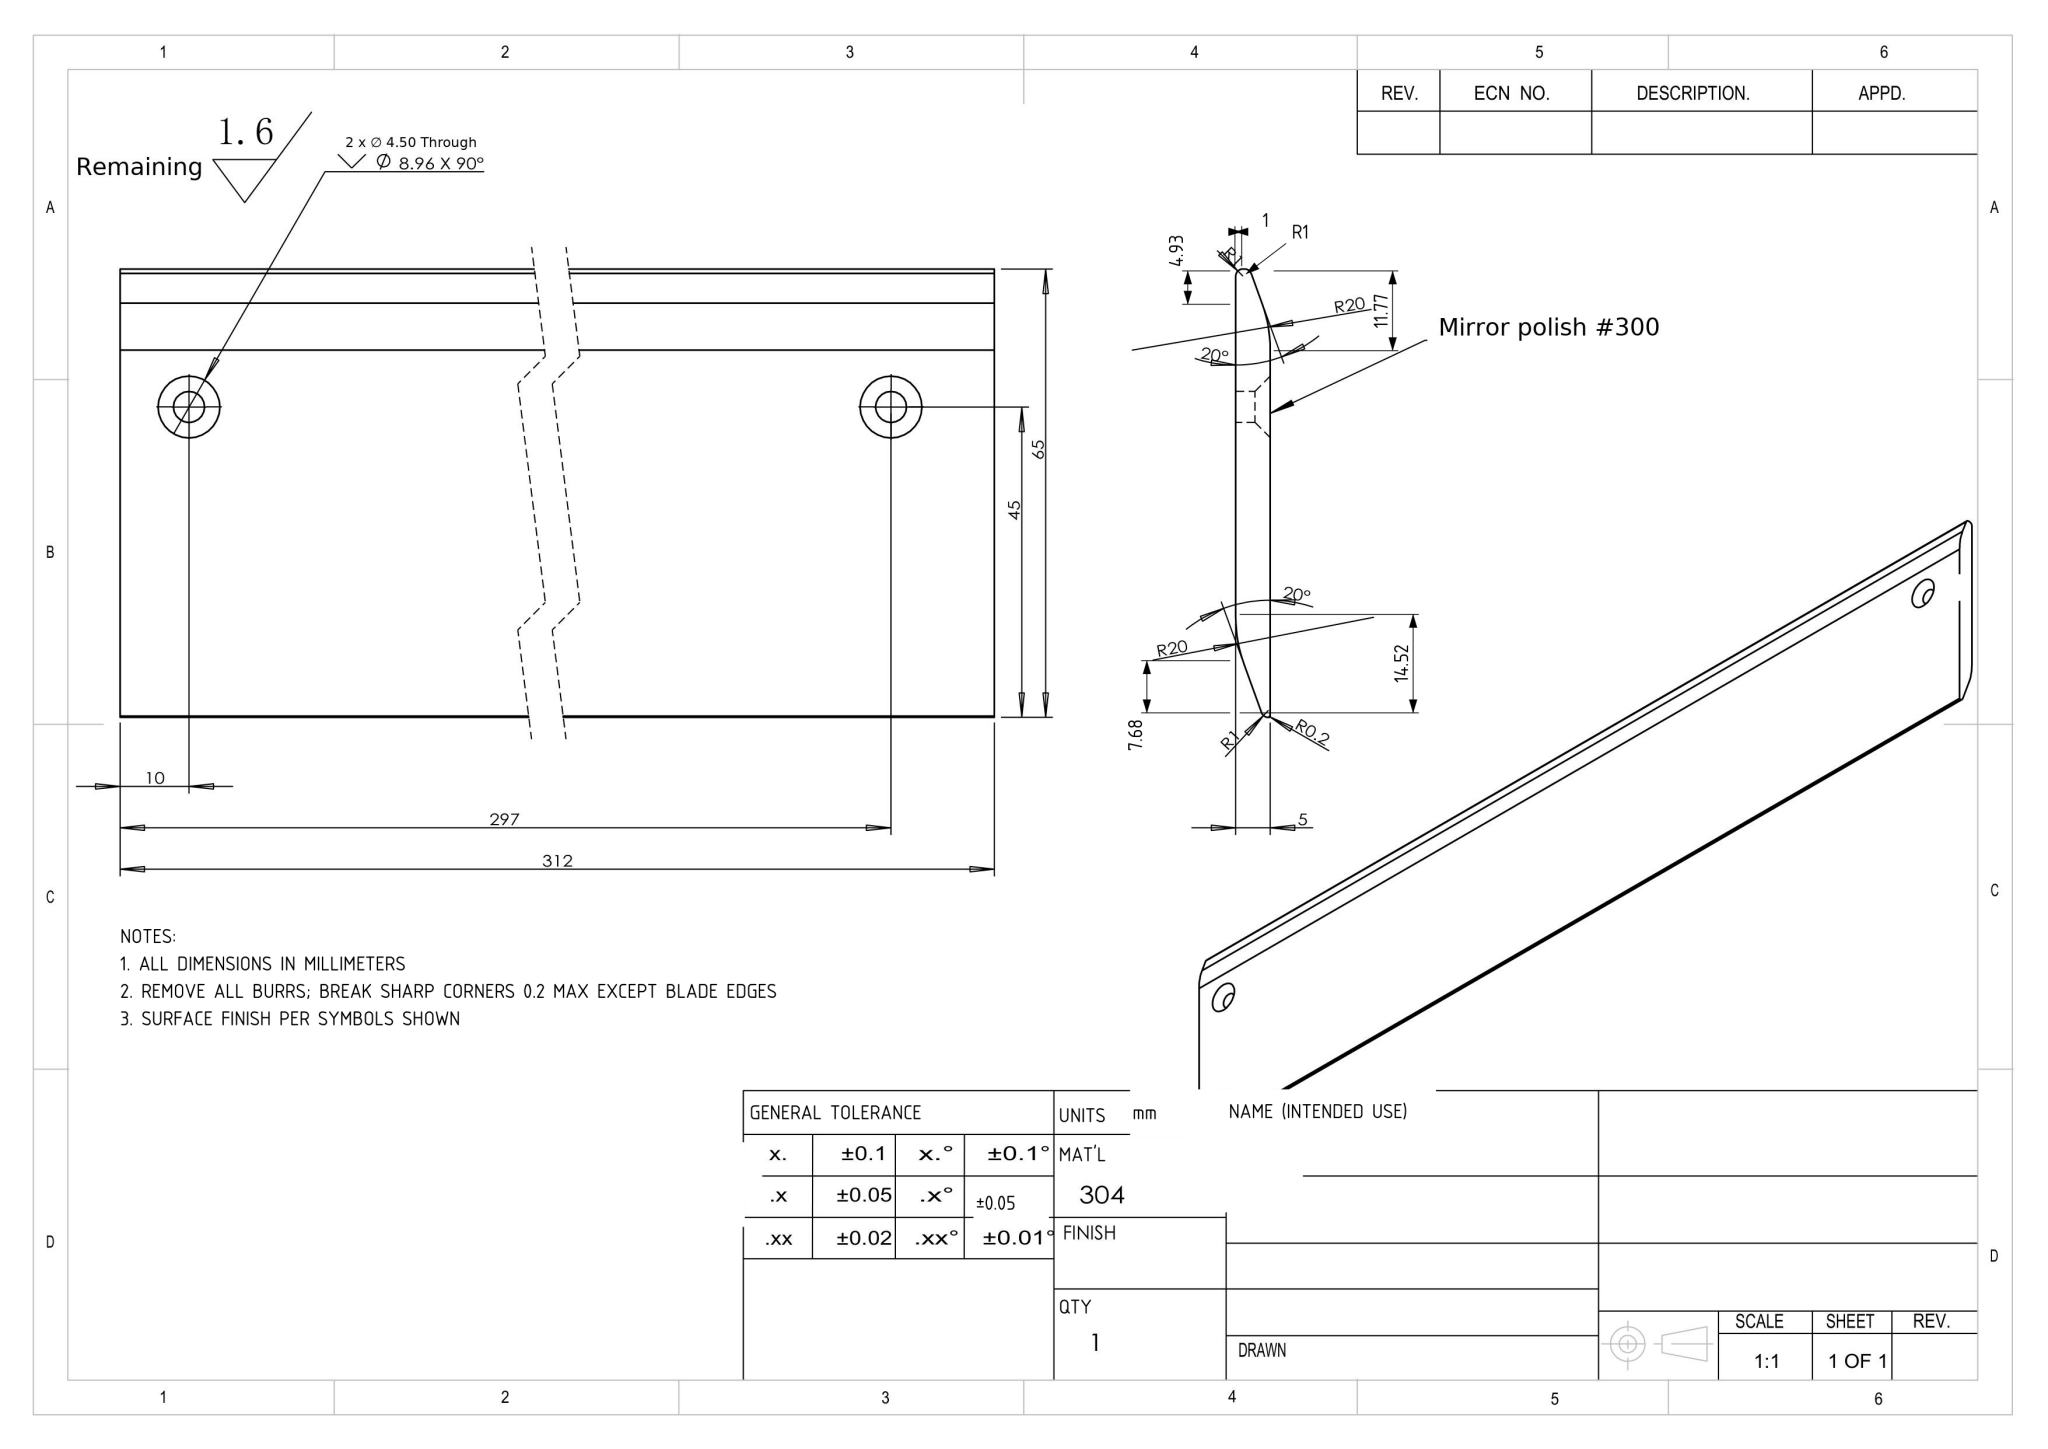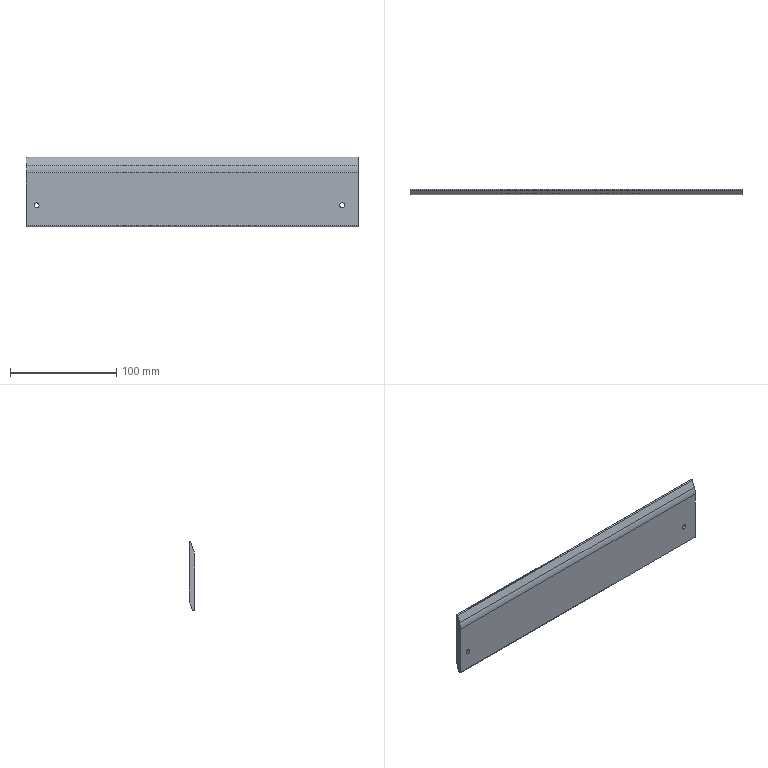Part | NX | mm | 1 solid | 22 faces | box 312 x 5 x 65 mm | volume 89859 mm3 | cylinder 10 | plane 8 | cone 4 | commonest cylinder face diameters 4.5 x4 2 x3 40 x2 0.4 x1
STEP:
#1=CARTESIAN_POINT('',(297.,2.77,-47.25));
#2=VERTEX_POINT('',#1);
#3=CARTESIAN_POINT('',(297.,2.77,-42.75));
#4=VERTEX_POINT('',#3);
#5=CARTESIAN_POINT('',(297.,2.77,-45.));
#6=DIRECTION('',(0.,1.,0.));
#7=DIRECTION('',(0.,0.,1.));
#8=AXIS2_PLACEMENT_3D('',#5,#6,#7);
#9=CIRCLE('',#8,2.25);
#10=EDGE_CURVE('',#2,#4,#9,.T.);
#11=ORIENTED_EDGE('',*,*,#10,.F.);
#12=CARTESIAN_POINT('',(297.,5.,-49.48));
#13=VERTEX_POINT('',#12);
#14=CARTESIAN_POINT('',(297.,5.,-49.48));
#15=DIRECTION('',(0.,0.7071,-0.7071));
#16=VECTOR('',#15,1000.);
#17=LINE('',#14,#16);
#18=EDGE_CURVE('',#2,#13,#17,.T.);
#19=ORIENTED_EDGE('',*,*,#18,.T.);
#20=CARTESIAN_POINT('',(297.,5.,-40.52));
#21=VERTEX_POINT('',#20);
#22=CARTESIAN_POINT('',(297.,5.,-45.));
#23=DIRECTION('',(0.,1.,0.));
#24=DIRECTION('',(0.,0.,1.));
#25=AXIS2_PLACEMENT_3D('',#22,#23,#24);
#26=CIRCLE('',#25,4.48);
#27=EDGE_CURVE('',#13,#21,#26,.T.);
#28=ORIENTED_EDGE('',*,*,#27,.T.);
#29=CARTESIAN_POINT('',(297.,5.,-40.52));
#30=DIRECTION('',(0.,0.7071,0.7071));
#31=VECTOR('',#30,1000.);
#32=LINE('',#29,#31);
#33=EDGE_CURVE('',#4,#21,#32,.T.);
#34=ORIENTED_EDGE('',*,*,#33,.F.);
#35=EDGE_LOOP('',(#11,#19,#28,#34));
#36=FACE_OUTER_BOUND('',#35,.T.);
#37=CARTESIAN_POINT('',(297.,5.,-45.));
#38=DIRECTION('',(0.,1.,0.));
#39=DIRECTION('',(0.,0.,1.));
#40=AXIS2_PLACEMENT_3D('',#37,#38,#39);
#41=CONICAL_SURFACE('',#40,4.48,0.7854);
#42=ADVANCED_FACE('',(#36),#41,.F.);
#43=CARTESIAN_POINT('',(297.,0.,-42.75));
#44=VERTEX_POINT('',#43);
#45=CARTESIAN_POINT('',(297.,0.,-47.25));
#46=VERTEX_POINT('',#45);
#47=CARTESIAN_POINT('',(297.,0.,-45.));
#48=DIRECTION('',(0.,-1.,0.));
#49=DIRECTION('',(0.,0.,-1.));
#50=AXIS2_PLACEMENT_3D('',#47,#48,#49);
#51=CIRCLE('',#50,2.25);
#52=EDGE_CURVE('',#44,#46,#51,.T.);
#53=ORIENTED_EDGE('',*,*,#52,.T.);
#54=CARTESIAN_POINT('',(297.,5.,-47.25));
#55=DIRECTION('',(0.,1.,0.));
#56=VECTOR('',#55,1000.);
#57=LINE('',#54,#56);
#58=EDGE_CURVE('',#46,#2,#57,.T.);
#59=ORIENTED_EDGE('',*,*,#58,.T.);
#60=ORIENTED_EDGE('',*,*,#10,.T.);
#61=CARTESIAN_POINT('',(297.,5.,-42.75));
#62=DIRECTION('',(0.,1.,0.));
#63=VECTOR('',#62,1000.);
#64=LINE('',#61,#63);
#65=EDGE_CURVE('',#44,#4,#64,.T.);
#66=ORIENTED_EDGE('',*,*,#65,.F.);
#67=EDGE_LOOP('',(#53,#59,#60,#66));
#68=FACE_OUTER_BOUND('',#67,.T.);
#69=CARTESIAN_POINT('',(297.,5.,-45.));
#70=DIRECTION('',(0.,1.,0.));
#71=DIRECTION('',(0.,0.,1.));
#72=AXIS2_PLACEMENT_3D('',#69,#70,#71);
#73=CYLINDRICAL_SURFACE('',#72,2.25);
#74=ADVANCED_FACE('',(#68),#73,.F.);
#75=CARTESIAN_POINT('',(10.,2.77,-47.25));
#76=VERTEX_POINT('',#75);
#77=CARTESIAN_POINT('',(10.,2.77,-42.75));
#78=VERTEX_POINT('',#77);
#79=CARTESIAN_POINT('',(10.,2.77,-45.));
#80=DIRECTION('',(0.,1.,0.));
#81=DIRECTION('',(0.,0.,1.));
#82=AXIS2_PLACEMENT_3D('',#79,#80,#81);
#83=CIRCLE('',#82,2.25);
#84=EDGE_CURVE('',#76,#78,#83,.T.);
#85=ORIENTED_EDGE('',*,*,#84,.F.);
#86=CARTESIAN_POINT('',(10.,5.,-49.48));
#87=VERTEX_POINT('',#86);
#88=CARTESIAN_POINT('',(10.,5.,-49.48));
#89=DIRECTION('',(0.,0.7071,-0.7071));
#90=VECTOR('',#89,1000.);
#91=LINE('',#88,#90);
#92=EDGE_CURVE('',#76,#87,#91,.T.);
#93=ORIENTED_EDGE('',*,*,#92,.T.);
#94=CARTESIAN_POINT('',(10.,5.,-40.52));
#95=VERTEX_POINT('',#94);
#96=CARTESIAN_POINT('',(10.,5.,-45.));
#97=DIRECTION('',(0.,1.,0.));
#98=DIRECTION('',(0.,0.,1.));
#99=AXIS2_PLACEMENT_3D('',#96,#97,#98);
#100=CIRCLE('',#99,4.48);
#101=EDGE_CURVE('',#87,#95,#100,.T.);
#102=ORIENTED_EDGE('',*,*,#101,.T.);
#103=CARTESIAN_POINT('',(10.,5.,-40.52));
#104=DIRECTION('',(0.,0.7071,0.7071));
#105=VECTOR('',#104,1000.);
#106=LINE('',#103,#105);
#107=EDGE_CURVE('',#78,#95,#106,.T.);
#108=ORIENTED_EDGE('',*,*,#107,.F.);
#109=EDGE_LOOP('',(#85,#93,#102,#108));
#110=FACE_OUTER_BOUND('',#109,.T.);
#111=CARTESIAN_POINT('',(10.,5.,-45.));
#112=DIRECTION('',(0.,1.,0.));
#113=DIRECTION('',(0.,0.,1.));
#114=AXIS2_PLACEMENT_3D('',#111,#112,#113);
#115=CONICAL_SURFACE('',#114,4.48,0.7854);
#116=ADVANCED_FACE('',(#110),#115,.F.);
#117=CARTESIAN_POINT('',(10.,0.,-42.75));
#118=VERTEX_POINT('',#117);
#119=CARTESIAN_POINT('',(10.,0.,-47.25));
#120=VERTEX_POINT('',#119);
#121=CARTESIAN_POINT('',(10.,0.,-45.));
#122=DIRECTION('',(0.,-1.,0.));
#123=DIRECTION('',(0.,0.,-1.));
#124=AXIS2_PLACEMENT_3D('',#121,#122,#123);
#125=CIRCLE('',#124,2.25);
#126=EDGE_CURVE('',#118,#120,#125,.T.);
#127=ORIENTED_EDGE('',*,*,#126,.T.);
#128=CARTESIAN_POINT('',(10.,5.,-47.25));
#129=DIRECTION('',(0.,1.,0.));
#130=VECTOR('',#129,1000.);
#131=LINE('',#128,#130);
#132=EDGE_CURVE('',#120,#76,#131,.T.);
#133=ORIENTED_EDGE('',*,*,#132,.T.);
#134=ORIENTED_EDGE('',*,*,#84,.T.);
#135=CARTESIAN_POINT('',(10.,5.,-42.75));
#136=DIRECTION('',(0.,1.,0.));
#137=VECTOR('',#136,1000.);
#138=LINE('',#135,#137);
#139=EDGE_CURVE('',#118,#78,#138,.T.);
#140=ORIENTED_EDGE('',*,*,#139,.F.);
#141=EDGE_LOOP('',(#127,#133,#134,#140));
#142=FACE_OUTER_BOUND('',#141,.T.);
#143=CARTESIAN_POINT('',(10.,5.,-45.));
#144=DIRECTION('',(0.,1.,0.));
#145=DIRECTION('',(0.,0.,1.));
#146=AXIS2_PLACEMENT_3D('',#143,#144,#145);
#147=CYLINDRICAL_SURFACE('',#146,2.25);
#148=ADVANCED_FACE('',(#142),#147,.F.);
#149=CARTESIAN_POINT('',(10.,5.,-45.));
#150=DIRECTION('',(0.,1.,0.));
#151=DIRECTION('',(0.,0.,1.));
#152=AXIS2_PLACEMENT_3D('',#149,#150,#151);
#153=CIRCLE('',#152,4.48);
#154=EDGE_CURVE('',#95,#87,#153,.T.);
#155=ORIENTED_EDGE('',*,*,#154,.F.);
#156=ORIENTED_EDGE('',*,*,#101,.F.);
#157=EDGE_LOOP('',(#155,#156));
#158=FACE_BOUND('',#157,.T.);
#159=CARTESIAN_POINT('',(0.,5.,-0.2));
#160=VERTEX_POINT('',#159);
#161=CARTESIAN_POINT('',(312.,5.,-0.2));
#162=VERTEX_POINT('',#161);
#163=CARTESIAN_POINT('',(0.,5.,-0.2));
#164=DIRECTION('',(1.,0.,0.));
#165=VECTOR('',#164,1000.);
#166=LINE('',#163,#165);
#167=EDGE_CURVE('',#160,#162,#166,.T.);
#168=ORIENTED_EDGE('',*,*,#167,.T.);
#169=CARTESIAN_POINT('',(312.,5.,-53.231));
#170=VERTEX_POINT('',#169);
#171=CARTESIAN_POINT('',(312.,5.,-0.));
#172=DIRECTION('',(0.,0.,1.));
#173=VECTOR('',#172,1000.);
#174=LINE('',#171,#173);
#175=EDGE_CURVE('',#170,#162,#174,.T.);
#176=ORIENTED_EDGE('',*,*,#175,.F.);
#177=CARTESIAN_POINT('',(0.,5.,-53.231));
#178=VERTEX_POINT('',#177);
#179=CARTESIAN_POINT('',(0.,5.,-53.231));
#180=DIRECTION('',(-1.,0.,0.));
#181=VECTOR('',#180,1000.);
#182=LINE('',#179,#181);
#183=EDGE_CURVE('',#170,#178,#182,.T.);
#184=ORIENTED_EDGE('',*,*,#183,.T.);
#185=CARTESIAN_POINT('',(0.,5.,0.));
#186=DIRECTION('',(0.,0.,1.));
#187=VECTOR('',#186,1000.);
#188=LINE('',#185,#187);
#189=EDGE_CURVE('',#178,#160,#188,.T.);
#190=ORIENTED_EDGE('',*,*,#189,.T.);
#191=EDGE_LOOP('',(#168,#176,#184,#190));
#192=FACE_OUTER_BOUND('',#191,.T.);
#193=CARTESIAN_POINT('',(297.,5.,-45.));
#194=DIRECTION('',(0.,1.,0.));
#195=DIRECTION('',(0.,0.,1.));
#196=AXIS2_PLACEMENT_3D('',#193,#194,#195);
#197=CIRCLE('',#196,4.48);
#198=EDGE_CURVE('',#21,#13,#197,.T.);
#199=ORIENTED_EDGE('',*,*,#198,.F.);
#200=ORIENTED_EDGE('',*,*,#27,.F.);
#201=EDGE_LOOP('',(#199,#200));
#202=FACE_BOUND('',#201,.T.);
#203=CARTESIAN_POINT('',(0.,5.,0.));
#204=DIRECTION('',(0.,-1.,0.));
#205=DIRECTION('',(0.,0.,-1.));
#206=AXIS2_PLACEMENT_3D('',#203,#204,#205);
#207=PLANE('',#206);
#208=ADVANCED_FACE('',(#158,#192,#202),#207,.F.);
#209=CARTESIAN_POINT('',(0.,4.8,0.));
#210=VERTEX_POINT('',#209);
#211=CARTESIAN_POINT('',(0.,4.7,0.));
#212=VERTEX_POINT('',#211);
#213=CARTESIAN_POINT('',(0.,5.,0.));
#214=DIRECTION('',(0.,-1.,0.));
#215=VECTOR('',#214,1000.);
#216=LINE('',#213,#215);
#217=EDGE_CURVE('',#210,#212,#216,.T.);
#218=ORIENTED_EDGE('',*,*,#217,.F.);
#219=CARTESIAN_POINT('',(0.,4.8,-0.2));
#220=DIRECTION('',(-1.,0.,0.));
#221=DIRECTION('',(0.,0.,-1.));
#222=AXIS2_PLACEMENT_3D('',#219,#220,#221);
#223=CIRCLE('',#222,0.2);
#224=EDGE_CURVE('',#210,#160,#223,.T.);
#225=ORIENTED_EDGE('',*,*,#224,.T.);
#226=ORIENTED_EDGE('',*,*,#189,.F.);
#227=CARTESIAN_POINT('',(0.,3.794,-60.071));
#228=VERTEX_POINT('',#227);
#229=CARTESIAN_POINT('',(0.,-15.,-53.231));
#230=DIRECTION('',(-1.,0.,0.));
#231=DIRECTION('',(0.,-0.,-1.));
#232=AXIS2_PLACEMENT_3D('',#229,#230,#231);
#233=CIRCLE('',#232,20.);
#234=EDGE_CURVE('',#178,#228,#233,.T.);
#235=ORIENTED_EDGE('',*,*,#234,.T.);
#236=CARTESIAN_POINT('',(0.,2.239,-64.342));
#237=VERTEX_POINT('',#236);
#238=CARTESIAN_POINT('',(0.,5.,-56.758));
#239=DIRECTION('',(0.,-0.342,-0.9397));
#240=VECTOR('',#239,1000.);
#241=LINE('',#238,#240);
#242=EDGE_CURVE('',#228,#237,#241,.T.);
#243=ORIENTED_EDGE('',*,*,#242,.T.);
#244=CARTESIAN_POINT('',(0.,1.3,-65.));
#245=VERTEX_POINT('',#244);
#246=CARTESIAN_POINT('',(0.,1.3,-64.));
#247=DIRECTION('',(-1.,0.,0.));
#248=DIRECTION('',(0.,0.,-1.));
#249=AXIS2_PLACEMENT_3D('',#246,#247,#248);
#250=CIRCLE('',#249,1.);
#251=EDGE_CURVE('',#237,#245,#250,.T.);
#252=ORIENTED_EDGE('',*,*,#251,.T.);
#253=CARTESIAN_POINT('',(0.,1.,-65.));
#254=VERTEX_POINT('',#253);
#255=CARTESIAN_POINT('',(0.,5.,-65.));
#256=DIRECTION('',(0.,-1.,0.));
#257=VECTOR('',#256,1000.);
#258=LINE('',#255,#257);
#259=EDGE_CURVE('',#245,#254,#258,.T.);
#260=ORIENTED_EDGE('',*,*,#259,.T.);
#261=CARTESIAN_POINT('',(0.,0.,-64.));
#262=VERTEX_POINT('',#261);
#263=CARTESIAN_POINT('',(0.,1.,-64.));
#264=DIRECTION('',(-1.,0.,0.));
#265=DIRECTION('',(0.,0.,-1.));
#266=AXIS2_PLACEMENT_3D('',#263,#264,#265);
#267=CIRCLE('',#266,1.);
#268=EDGE_CURVE('',#254,#262,#267,.T.);
#269=ORIENTED_EDGE('',*,*,#268,.T.);
#270=CARTESIAN_POINT('',(0.,0.,-14.516));
#271=VERTEX_POINT('',#270);
#272=CARTESIAN_POINT('',(0.,0.,0.));
#273=DIRECTION('',(0.,0.,1.));
#274=VECTOR('',#273,1000.);
#275=LINE('',#272,#274);
#276=EDGE_CURVE('',#262,#271,#275,.T.);
#277=ORIENTED_EDGE('',*,*,#276,.T.);
#278=CARTESIAN_POINT('',(0.,1.206,-7.676));
#279=VERTEX_POINT('',#278);
#280=CARTESIAN_POINT('',(0.,20.,-14.516));
#281=DIRECTION('',(-1.,0.,0.));
#282=DIRECTION('',(0.,0.,-1.));
#283=AXIS2_PLACEMENT_3D('',#280,#281,#282);
#284=CIRCLE('',#283,20.);
#285=EDGE_CURVE('',#271,#279,#284,.T.);
#286=ORIENTED_EDGE('',*,*,#285,.T.);
#287=CARTESIAN_POINT('',(0.,3.761,-0.658));
#288=VERTEX_POINT('',#287);
#289=CARTESIAN_POINT('',(0.,4.,0.));
#290=DIRECTION('',(0.,0.342,0.9397));
#291=VECTOR('',#290,1000.);
#292=LINE('',#289,#291);
#293=EDGE_CURVE('',#279,#288,#292,.T.);
#294=ORIENTED_EDGE('',*,*,#293,.T.);
#295=CARTESIAN_POINT('',(0.,4.7,-1.));
#296=DIRECTION('',(-1.,0.,0.));
#297=DIRECTION('',(0.,0.,-1.));
#298=AXIS2_PLACEMENT_3D('',#295,#296,#297);
#299=CIRCLE('',#298,1.);
#300=EDGE_CURVE('',#288,#212,#299,.T.);
#301=ORIENTED_EDGE('',*,*,#300,.T.);
#302=EDGE_LOOP('',(#218,#225,#226,#235,#243,#252,#260,#269,#277,#286,#294,#301));
#303=FACE_OUTER_BOUND('',#302,.T.);
#304=CARTESIAN_POINT('',(0.,5.,0.));
#305=DIRECTION('',(1.,0.,0.));
#306=DIRECTION('',(0.,0.,-1.));
#307=AXIS2_PLACEMENT_3D('',#304,#305,#306);
#308=PLANE('',#307);
#309=ADVANCED_FACE('',(#303),#308,.F.);
#310=CARTESIAN_POINT('',(312.,4.7,-0.));
#311=VERTEX_POINT('',#310);
#312=CARTESIAN_POINT('',(342.,4.7,0.));
#313=DIRECTION('',(1.,0.,0.));
#314=VECTOR('',#313,1000.);
#315=LINE('',#312,#314);
#316=EDGE_CURVE('',#212,#311,#315,.T.);
#317=ORIENTED_EDGE('',*,*,#316,.T.);
#318=CARTESIAN_POINT('',(312.,4.8,-0.));
#319=VERTEX_POINT('',#318);
#320=CARTESIAN_POINT('',(312.,-5.,-0.));
#321=DIRECTION('',(0.,1.,0.));
#322=VECTOR('',#321,1000.);
#323=LINE('',#320,#322);
#324=EDGE_CURVE('',#311,#319,#323,.T.);
#325=ORIENTED_EDGE('',*,*,#324,.T.);
#326=CARTESIAN_POINT('',(0.,4.8,0.));
#327=DIRECTION('',(-1.,0.,0.));
#328=VECTOR('',#327,1000.);
#329=LINE('',#326,#328);
#330=EDGE_CURVE('',#319,#210,#329,.T.);
#331=ORIENTED_EDGE('',*,*,#330,.T.);
#332=ORIENTED_EDGE('',*,*,#217,.T.);
#333=EDGE_LOOP('',(#317,#325,#331,#332));
#334=FACE_OUTER_BOUND('',#333,.T.);
#335=CARTESIAN_POINT('',(0.,5.,0.));
#336=DIRECTION('',(0.,0.,-1.));
#337=DIRECTION('',(-1.,0.,0.));
#338=AXIS2_PLACEMENT_3D('',#335,#336,#337);
#339=PLANE('',#338);
#340=ADVANCED_FACE('',(#334),#339,.F.);
#341=CARTESIAN_POINT('',(312.,1.3,-65.));
#342=VERTEX_POINT('',#341);
#343=CARTESIAN_POINT('',(342.,1.3,-65.));
#344=DIRECTION('',(1.,0.,0.));
#345=VECTOR('',#344,1000.);
#346=LINE('',#343,#345);
#347=EDGE_CURVE('',#245,#342,#346,.T.);
#348=ORIENTED_EDGE('',*,*,#347,.T.);
#349=CARTESIAN_POINT('',(312.,1.,-65.));
#350=VERTEX_POINT('',#349);
#351=CARTESIAN_POINT('',(312.,5.,-65.));
#352=DIRECTION('',(0.,-1.,0.));
#353=VECTOR('',#352,1000.);
#354=LINE('',#351,#353);
#355=EDGE_CURVE('',#342,#350,#354,.T.);
#356=ORIENTED_EDGE('',*,*,#355,.T.);
#357=CARTESIAN_POINT('',(0.,1.,-65.));
#358=DIRECTION('',(-1.,0.,0.));
#359=VECTOR('',#358,1000.);
#360=LINE('',#357,#359);
#361=EDGE_CURVE('',#350,#254,#360,.T.);
#362=ORIENTED_EDGE('',*,*,#361,.T.);
#363=ORIENTED_EDGE('',*,*,#259,.F.);
#364=EDGE_LOOP('',(#348,#356,#362,#363));
#365=FACE_OUTER_BOUND('',#364,.T.);
#366=CARTESIAN_POINT('',(0.,5.,-65.));
#367=DIRECTION('',(0.,0.,1.));
#368=DIRECTION('',(1.,0.,0.));
#369=AXIS2_PLACEMENT_3D('',#366,#367,#368);
#370=PLANE('',#369);
#371=ADVANCED_FACE('',(#365),#370,.F.);
#372=CARTESIAN_POINT('',(312.,0.,-14.516));
#373=VERTEX_POINT('',#372);
#374=CARTESIAN_POINT('',(312.,0.,-64.));
#375=VERTEX_POINT('',#374);
#376=CARTESIAN_POINT('',(312.,0.,0.));
#377=DIRECTION('',(0.,0.,-1.));
#378=VECTOR('',#377,1000.);
#379=LINE('',#376,#378);
#380=EDGE_CURVE('',#373,#375,#379,.T.);
#381=ORIENTED_EDGE('',*,*,#380,.F.);
#382=CARTESIAN_POINT('',(0.,0.,-14.516));
#383=DIRECTION('',(-1.,0.,0.));
#384=VECTOR('',#383,1000.);
#385=LINE('',#382,#384);
#386=EDGE_CURVE('',#373,#271,#385,.T.);
#387=ORIENTED_EDGE('',*,*,#386,.T.);
#388=ORIENTED_EDGE('',*,*,#276,.F.);
#389=CARTESIAN_POINT('',(342.,0.,-64.));
#390=DIRECTION('',(1.,0.,0.));
#391=VECTOR('',#390,1000.);
#392=LINE('',#389,#391);
#393=EDGE_CURVE('',#262,#375,#392,.T.);
#394=ORIENTED_EDGE('',*,*,#393,.T.);
#395=EDGE_LOOP('',(#381,#387,#388,#394));
#396=FACE_OUTER_BOUND('',#395,.T.);
#397=ORIENTED_EDGE('',*,*,#52,.F.);
#398=CARTESIAN_POINT('',(297.,0.,-45.));
#399=DIRECTION('',(0.,-1.,0.));
#400=DIRECTION('',(0.,0.,-1.));
#401=AXIS2_PLACEMENT_3D('',#398,#399,#400);
#402=CIRCLE('',#401,2.25);
#403=EDGE_CURVE('',#46,#44,#402,.T.);
#404=ORIENTED_EDGE('',*,*,#403,.F.);
#405=EDGE_LOOP('',(#397,#404));
#406=FACE_BOUND('',#405,.T.);
#407=ORIENTED_EDGE('',*,*,#126,.F.);
#408=CARTESIAN_POINT('',(10.,0.,-45.));
#409=DIRECTION('',(0.,-1.,0.));
#410=DIRECTION('',(0.,0.,-1.));
#411=AXIS2_PLACEMENT_3D('',#408,#409,#410);
#412=CIRCLE('',#411,2.25);
#413=EDGE_CURVE('',#120,#118,#412,.T.);
#414=ORIENTED_EDGE('',*,*,#413,.F.);
#415=EDGE_LOOP('',(#407,#414));
#416=FACE_BOUND('',#415,.T.);
#417=CARTESIAN_POINT('',(0.,0.,0.));
#418=DIRECTION('',(0.,-1.,0.));
#419=DIRECTION('',(0.,0.,-1.));
#420=AXIS2_PLACEMENT_3D('',#417,#418,#419);
#421=PLANE('',#420);
#422=ADVANCED_FACE('',(#396,#406,#416),#421,.T.);
#423=CARTESIAN_POINT('',(312.,2.239,-64.342));
#424=VERTEX_POINT('',#423);
#425=CARTESIAN_POINT('',(312.,3.794,-60.071));
#426=VERTEX_POINT('',#425);
#427=CARTESIAN_POINT('',(312.,5.,-56.758));
#428=DIRECTION('',(0.,0.342,0.9397));
#429=VECTOR('',#428,1000.);
#430=LINE('',#427,#429);
#431=EDGE_CURVE('',#424,#426,#430,.T.);
#432=ORIENTED_EDGE('',*,*,#431,.F.);
#433=CARTESIAN_POINT('',(0.,2.239,-64.342));
#434=DIRECTION('',(-1.,0.,0.));
#435=VECTOR('',#434,1000.);
#436=LINE('',#433,#435);
#437=EDGE_CURVE('',#424,#237,#436,.T.);
#438=ORIENTED_EDGE('',*,*,#437,.T.);
#439=ORIENTED_EDGE('',*,*,#242,.F.);
#440=CARTESIAN_POINT('',(342.,3.794,-60.071));
#441=DIRECTION('',(1.,0.,0.));
#442=VECTOR('',#441,1000.);
#443=LINE('',#440,#442);
#444=EDGE_CURVE('',#228,#426,#443,.T.);
#445=ORIENTED_EDGE('',*,*,#444,.T.);
#446=EDGE_LOOP('',(#432,#438,#439,#445));
#447=FACE_OUTER_BOUND('',#446,.T.);
#448=CARTESIAN_POINT('',(0.,5.,-56.758));
#449=DIRECTION('',(0.,-0.9397,0.342));
#450=DIRECTION('',(-1.,0.,0.));
#451=AXIS2_PLACEMENT_3D('',#448,#449,#450);
#452=PLANE('',#451);
#453=ADVANCED_FACE('',(#447),#452,.F.);
#454=CARTESIAN_POINT('',(312.,1.,-64.));
#455=DIRECTION('',(1.,0.,0.));
#456=DIRECTION('',(0.,0.,1.));
#457=AXIS2_PLACEMENT_3D('',#454,#455,#456);
#458=CIRCLE('',#457,1.);
#459=EDGE_CURVE('',#375,#350,#458,.T.);
#460=ORIENTED_EDGE('',*,*,#459,.F.);
#461=ORIENTED_EDGE('',*,*,#393,.F.);
#462=ORIENTED_EDGE('',*,*,#268,.F.);
#463=ORIENTED_EDGE('',*,*,#361,.F.);
#464=EDGE_LOOP('',(#460,#461,#462,#463));
#465=FACE_OUTER_BOUND('',#464,.T.);
#466=CARTESIAN_POINT('',(0.,1.,-64.));
#467=DIRECTION('',(1.,0.,0.));
#468=DIRECTION('',(0.,0.,-1.));
#469=AXIS2_PLACEMENT_3D('',#466,#467,#468);
#470=CYLINDRICAL_SURFACE('',#469,1.);
#471=ADVANCED_FACE('',(#465),#470,.T.);
#472=CARTESIAN_POINT('',(312.,1.3,-64.));
#473=DIRECTION('',(1.,0.,0.));
#474=DIRECTION('',(0.,0.,1.));
#475=AXIS2_PLACEMENT_3D('',#472,#473,#474);
#476=CIRCLE('',#475,1.);
#477=EDGE_CURVE('',#342,#424,#476,.T.);
#478=ORIENTED_EDGE('',*,*,#477,.F.);
#479=ORIENTED_EDGE('',*,*,#347,.F.);
#480=ORIENTED_EDGE('',*,*,#251,.F.);
#481=ORIENTED_EDGE('',*,*,#437,.F.);
#482=EDGE_LOOP('',(#478,#479,#480,#481));
#483=FACE_OUTER_BOUND('',#482,.T.);
#484=CARTESIAN_POINT('',(0.,1.3,-64.));
#485=DIRECTION('',(1.,0.,0.));
#486=DIRECTION('',(0.,0.,-1.));
#487=AXIS2_PLACEMENT_3D('',#484,#485,#486);
#488=CYLINDRICAL_SURFACE('',#487,1.);
#489=ADVANCED_FACE('',(#483),#488,.T.);
#490=CARTESIAN_POINT('',(312.,-15.,-53.231));
#491=DIRECTION('',(1.,0.,0.));
#492=DIRECTION('',(0.,-0.,1.));
#493=AXIS2_PLACEMENT_3D('',#490,#491,#492);
#494=CIRCLE('',#493,20.);
#495=EDGE_CURVE('',#426,#170,#494,.T.);
#496=ORIENTED_EDGE('',*,*,#495,.F.);
#497=ORIENTED_EDGE('',*,*,#444,.F.);
#498=ORIENTED_EDGE('',*,*,#234,.F.);
#499=ORIENTED_EDGE('',*,*,#183,.F.);
#500=EDGE_LOOP('',(#496,#497,#498,#499));
#501=FACE_OUTER_BOUND('',#500,.T.);
#502=CARTESIAN_POINT('',(0.,-15.,-53.231));
#503=DIRECTION('',(-1.,0.,0.));
#504=DIRECTION('',(0.,0.,1.));
#505=AXIS2_PLACEMENT_3D('',#502,#503,#504);
#506=CYLINDRICAL_SURFACE('',#505,20.);
#507=ADVANCED_FACE('',(#501),#506,.T.);
#508=ORIENTED_EDGE('',*,*,#132,.F.);
#509=ORIENTED_EDGE('',*,*,#413,.T.);
#510=ORIENTED_EDGE('',*,*,#139,.T.);
#511=CARTESIAN_POINT('',(10.,2.77,-45.));
#512=DIRECTION('',(0.,1.,0.));
#513=DIRECTION('',(0.,0.,1.));
#514=AXIS2_PLACEMENT_3D('',#511,#512,#513);
#515=CIRCLE('',#514,2.25);
#516=EDGE_CURVE('',#78,#76,#515,.T.);
#517=ORIENTED_EDGE('',*,*,#516,.T.);
#518=EDGE_LOOP('',(#508,#509,#510,#517));
#519=FACE_OUTER_BOUND('',#518,.T.);
#520=CARTESIAN_POINT('',(10.,5.,-45.));
#521=DIRECTION('',(0.,1.,0.));
#522=DIRECTION('',(0.,0.,1.));
#523=AXIS2_PLACEMENT_3D('',#520,#521,#522);
#524=CYLINDRICAL_SURFACE('',#523,2.25);
#525=ADVANCED_FACE('',(#519),#524,.F.);
#526=ORIENTED_EDGE('',*,*,#92,.F.);
#527=ORIENTED_EDGE('',*,*,#516,.F.);
#528=ORIENTED_EDGE('',*,*,#107,.T.);
#529=ORIENTED_EDGE('',*,*,#154,.T.);
#530=EDGE_LOOP('',(#526,#527,#528,#529));
#531=FACE_OUTER_BOUND('',#530,.T.);
#532=CARTESIAN_POINT('',(10.,5.,-45.));
#533=DIRECTION('',(0.,1.,0.));
#534=DIRECTION('',(0.,0.,1.));
#535=AXIS2_PLACEMENT_3D('',#532,#533,#534);
#536=CONICAL_SURFACE('',#535,4.48,0.7854);
#537=ADVANCED_FACE('',(#531),#536,.F.);
#538=ORIENTED_EDGE('',*,*,#58,.F.);
#539=ORIENTED_EDGE('',*,*,#403,.T.);
#540=ORIENTED_EDGE('',*,*,#65,.T.);
#541=CARTESIAN_POINT('',(297.,2.77,-45.));
#542=DIRECTION('',(0.,1.,0.));
#543=DIRECTION('',(0.,0.,1.));
#544=AXIS2_PLACEMENT_3D('',#541,#542,#543);
#545=CIRCLE('',#544,2.25);
#546=EDGE_CURVE('',#4,#2,#545,.T.);
#547=ORIENTED_EDGE('',*,*,#546,.T.);
#548=EDGE_LOOP('',(#538,#539,#540,#547));
#549=FACE_OUTER_BOUND('',#548,.T.);
#550=CARTESIAN_POINT('',(297.,5.,-45.));
#551=DIRECTION('',(0.,1.,0.));
#552=DIRECTION('',(0.,0.,1.));
#553=AXIS2_PLACEMENT_3D('',#550,#551,#552);
#554=CYLINDRICAL_SURFACE('',#553,2.25);
#555=ADVANCED_FACE('',(#549),#554,.F.);
#556=ORIENTED_EDGE('',*,*,#18,.F.);
#557=ORIENTED_EDGE('',*,*,#546,.F.);
#558=ORIENTED_EDGE('',*,*,#33,.T.);
#559=ORIENTED_EDGE('',*,*,#198,.T.);
#560=EDGE_LOOP('',(#556,#557,#558,#559));
#561=FACE_OUTER_BOUND('',#560,.T.);
#562=CARTESIAN_POINT('',(297.,5.,-45.));
#563=DIRECTION('',(0.,1.,0.));
#564=DIRECTION('',(0.,0.,1.));
#565=AXIS2_PLACEMENT_3D('',#562,#563,#564);
#566=CONICAL_SURFACE('',#565,4.48,0.7854);
#567=ADVANCED_FACE('',(#561),#566,.F.);
#568=CARTESIAN_POINT('',(312.,3.761,-0.658));
#569=VERTEX_POINT('',#568);
#570=CARTESIAN_POINT('',(312.,1.206,-7.676));
#571=VERTEX_POINT('',#570);
#572=CARTESIAN_POINT('',(312.,4.,0.));
#573=DIRECTION('',(0.,-0.342,-0.9397));
#574=VECTOR('',#573,1000.);
#575=LINE('',#572,#574);
#576=EDGE_CURVE('',#569,#571,#575,.T.);
#577=ORIENTED_EDGE('',*,*,#576,.F.);
#578=CARTESIAN_POINT('',(0.,3.761,-0.658));
#579=DIRECTION('',(-1.,0.,0.));
#580=VECTOR('',#579,1000.);
#581=LINE('',#578,#580);
#582=EDGE_CURVE('',#569,#288,#581,.T.);
#583=ORIENTED_EDGE('',*,*,#582,.T.);
#584=ORIENTED_EDGE('',*,*,#293,.F.);
#585=CARTESIAN_POINT('',(0.,1.206,-7.676));
#586=DIRECTION('',(1.,0.,0.));
#587=VECTOR('',#586,1000.);
#588=LINE('',#585,#587);
#589=EDGE_CURVE('',#279,#571,#588,.T.);
#590=ORIENTED_EDGE('',*,*,#589,.T.);
#591=EDGE_LOOP('',(#577,#583,#584,#590));
#592=FACE_OUTER_BOUND('',#591,.T.);
#593=CARTESIAN_POINT('',(0.,4.,0.));
#594=DIRECTION('',(0.,-0.9397,0.342));
#595=DIRECTION('',(-1.,0.,0.));
#596=AXIS2_PLACEMENT_3D('',#593,#594,#595);
#597=PLANE('',#596);
#598=ADVANCED_FACE('',(#592),#597,.T.);
#599=CARTESIAN_POINT('',(312.,20.,-14.516));
#600=DIRECTION('',(1.,0.,0.));
#601=DIRECTION('',(0.,0.,1.));
#602=AXIS2_PLACEMENT_3D('',#599,#600,#601);
#603=CIRCLE('',#602,20.);
#604=EDGE_CURVE('',#571,#373,#603,.T.);
#605=ORIENTED_EDGE('',*,*,#604,.F.);
#606=ORIENTED_EDGE('',*,*,#589,.F.);
#607=ORIENTED_EDGE('',*,*,#285,.F.);
#608=ORIENTED_EDGE('',*,*,#386,.F.);
#609=EDGE_LOOP('',(#605,#606,#607,#608));
#610=FACE_OUTER_BOUND('',#609,.T.);
#611=CARTESIAN_POINT('',(0.,20.,-14.516));
#612=DIRECTION('',(-1.,0.,0.));
#613=DIRECTION('',(0.,0.,1.));
#614=AXIS2_PLACEMENT_3D('',#611,#612,#613);
#615=CYLINDRICAL_SURFACE('',#614,20.);
#616=ADVANCED_FACE('',(#610),#615,.T.);
#617=CARTESIAN_POINT('',(312.,4.7,-1.));
#618=DIRECTION('',(1.,0.,0.));
#619=DIRECTION('',(0.,0.,1.));
#620=AXIS2_PLACEMENT_3D('',#617,#618,#619);
#621=CIRCLE('',#620,1.);
#622=EDGE_CURVE('',#311,#569,#621,.T.);
#623=ORIENTED_EDGE('',*,*,#622,.F.);
#624=ORIENTED_EDGE('',*,*,#316,.F.);
#625=ORIENTED_EDGE('',*,*,#300,.F.);
#626=ORIENTED_EDGE('',*,*,#582,.F.);
#627=EDGE_LOOP('',(#623,#624,#625,#626));
#628=FACE_OUTER_BOUND('',#627,.T.);
#629=CARTESIAN_POINT('',(0.,4.7,-1.));
#630=DIRECTION('',(-1.,0.,0.));
#631=DIRECTION('',(0.,0.,1.));
#632=AXIS2_PLACEMENT_3D('',#629,#630,#631);
#633=CYLINDRICAL_SURFACE('',#632,1.);
#634=ADVANCED_FACE('',(#628),#633,.T.);
#635=CARTESIAN_POINT('',(312.,4.8,-0.2));
#636=DIRECTION('',(1.,0.,0.));
#637=DIRECTION('',(0.,0.,1.));
#638=AXIS2_PLACEMENT_3D('',#635,#636,#637);
#639=CIRCLE('',#638,0.2);
#640=EDGE_CURVE('',#162,#319,#639,.T.);
#641=ORIENTED_EDGE('',*,*,#640,.F.);
#642=ORIENTED_EDGE('',*,*,#167,.F.);
#643=ORIENTED_EDGE('',*,*,#224,.F.);
#644=ORIENTED_EDGE('',*,*,#330,.F.);
#645=EDGE_LOOP('',(#641,#642,#643,#644));
#646=FACE_OUTER_BOUND('',#645,.T.);
#647=CARTESIAN_POINT('',(0.,4.8,-0.2));
#648=DIRECTION('',(1.,0.,0.));
#649=DIRECTION('',(0.,0.,-1.));
#650=AXIS2_PLACEMENT_3D('',#647,#648,#649);
#651=CYLINDRICAL_SURFACE('',#650,0.2);
#652=ADVANCED_FACE('',(#646),#651,.T.);
#653=ORIENTED_EDGE('',*,*,#495,.T.);
#654=ORIENTED_EDGE('',*,*,#175,.T.);
#655=ORIENTED_EDGE('',*,*,#640,.T.);
#656=ORIENTED_EDGE('',*,*,#324,.F.);
#657=ORIENTED_EDGE('',*,*,#622,.T.);
#658=ORIENTED_EDGE('',*,*,#576,.T.);
#659=ORIENTED_EDGE('',*,*,#604,.T.);
#660=ORIENTED_EDGE('',*,*,#380,.T.);
#661=ORIENTED_EDGE('',*,*,#459,.T.);
#662=ORIENTED_EDGE('',*,*,#355,.F.);
#663=ORIENTED_EDGE('',*,*,#477,.T.);
#664=ORIENTED_EDGE('',*,*,#431,.T.);
#665=EDGE_LOOP('',(#653,#654,#655,#656,#657,#658,#659,#660,#661,#662,#663,#664));
#666=FACE_OUTER_BOUND('',#665,.T.);
#667=CARTESIAN_POINT('',(312.,-5.,-0.));
#668=DIRECTION('',(-1.,0.,0.));
#669=DIRECTION('',(0.,0.,1.));
#670=AXIS2_PLACEMENT_3D('',#667,#668,#669);
#671=PLANE('',#670);
#672=ADVANCED_FACE('',(#666),#671,.F.);
#673=CLOSED_SHELL('',(#42,#74,#116,#148,#208,#309,#340,#371,#422,#453,#471,#489,#507,#525,#537,#555,#567,#598,#616,#634,#652,#672));
#674=MANIFOLD_SOLID_BREP('',#673);
#675=CARTESIAN_POINT('',(0.,0.,0.));
#676=DIRECTION('',(0.,0.,1.));
#677=DIRECTION('',(1.,0.,0.));
#678=AXIS2_PLACEMENT_3D('',#675,#676,#677);
#679=(LENGTH_UNIT()NAMED_UNIT(*)SI_UNIT(.MILLI.,.METRE.));
#680=UNCERTAINTY_MEASURE_WITH_UNIT(LENGTH_MEASURE(0.00001),#679,'','');
#681=(NAMED_UNIT(*)PLANE_ANGLE_UNIT()SI_UNIT($,.RADIAN.));
#682=(NAMED_UNIT(*)SI_UNIT($,.STERADIAN.)SOLID_ANGLE_UNIT());
#683=(GEOMETRIC_REPRESENTATION_CONTEXT(3)GLOBAL_UNCERTAINTY_ASSIGNED_CONTEXT((#680))GLOBAL_UNIT_ASSIGNED_CONTEXT((#679,#681,#682))REPRESENTATION_CONTEXT('',''));
#684=ADVANCED_BREP_SHAPE_REPRESENTATION('',(#674,#678),#683);
#685=COLOUR_RGB('',0.7922,0.8196,0.9333);
#686=FILL_AREA_STYLE_COLOUR('',#685);
#687=FILL_AREA_STYLE('',(#686));
#688=SURFACE_STYLE_FILL_AREA(#687);
#689=SURFACE_SIDE_STYLE('',(#688));
#690=SURFACE_STYLE_USAGE(.BOTH.,#689);
#691=PRESENTATION_STYLE_ASSIGNMENT((#690));
#692=STYLED_ITEM('',(#691),#674);
#693=PRESENTATION_LAYER_ASSIGNMENT('','',(#692));
#694=(LENGTH_UNIT()NAMED_UNIT(*)SI_UNIT(.MILLI.,.METRE.));
#695=UNCERTAINTY_MEASURE_WITH_UNIT(LENGTH_MEASURE(0.00001),#694,'','');
#696=(NAMED_UNIT(*)PLANE_ANGLE_UNIT()SI_UNIT($,.RADIAN.));
#697=(NAMED_UNIT(*)SI_UNIT($,.STERADIAN.)SOLID_ANGLE_UNIT());
#698=(GEOMETRIC_REPRESENTATION_CONTEXT(3)GLOBAL_UNCERTAINTY_ASSIGNED_CONTEXT((#695))GLOBAL_UNIT_ASSIGNED_CONTEXT((#694,#696,#697))REPRESENTATION_CONTEXT('',''));
#699=MECHANICAL_DESIGN_GEOMETRIC_PRESENTATION_REPRESENTATION('',(#692),#698);